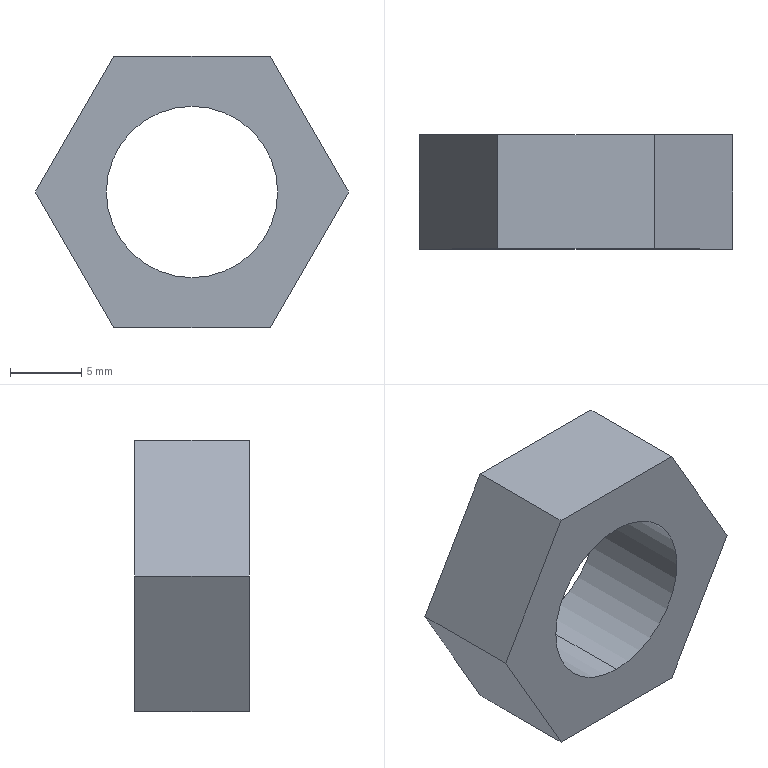Component | SolidWorks | M12Nut-1 | 1 solid | 10 faces | box 21.94 x 8 x 19 mm | volume 1596 mm3 | plane 8 | cylinder 2 | commonest cylinder face diameters 12 x2 | material #45
build123d program:
from build123d import *

# Parameters (mm, degrees)
BOSS_EXTRUDE1_DEPTH = 4
M12_TAPPED_HOLE1_D  = 12


with BuildPart() as part:
    # Sketch1 → Boss-Extrude1 (new, symmetric)
    with BuildSketch(Plane(origin=(0, 0, 0), x_dir=(1, 0, 0), z_dir=(0, 1, 0))):
        Polygon((5.485, 9.5), (-5.485, 9.5), (-10.97, 0), (-5.485, -9.5), (5.485, -9.5), (10.97, 0), align=None)
    extrude(amount=BOSS_EXTRUDE1_DEPTH, both=True)

    # M12 Tapped Hole1 (through all)
    with Locations(Plane(origin=(0, 4, 0), x_dir=(1, 0, 0), z_dir=(0, 1, 0))):
        with Locations((0, 0)):
            Hole(M12_TAPPED_HOLE1_D / 2)


solid = part.part

# Placed as in the assembly
solid = solid.moved(Location((40, -11.5, 60), (0, 0, 0)))
STEP:
#1=CARTESIAN_POINT('',(1.575,-0.6102,2.126));
#2=VERTEX_POINT('',#1);
#3=CARTESIAN_POINT('',(1.575,-0.6102,2.598));
#4=VERTEX_POINT('',#3);
#5=CARTESIAN_POINT('',(1.575,-0.6102,2.362));
#6=DIRECTION('',(0.,1.,0.));
#7=DIRECTION('',(0.,0.,1.));
#8=AXIS2_PLACEMENT_3D('',#5,#6,#7);
#9=CIRCLE('',#8,0.2362);
#10=EDGE_CURVE('',#2,#4,#9,.T.);
#11=ORIENTED_EDGE('',*,*,#10,.F.);
#12=CARTESIAN_POINT('',(1.575,-0.2953,2.126));
#13=VERTEX_POINT('',#12);
#14=CARTESIAN_POINT('',(1.575,-0.2953,2.126));
#15=DIRECTION('',(0.,1.,0.));
#16=VECTOR('',#15,39.37);
#17=LINE('',#14,#16);
#18=EDGE_CURVE('',#2,#13,#17,.T.);
#19=ORIENTED_EDGE('',*,*,#18,.T.);
#20=CARTESIAN_POINT('',(1.575,-0.2953,2.598));
#21=VERTEX_POINT('',#20);
#22=CARTESIAN_POINT('',(1.575,-0.2953,2.362));
#23=DIRECTION('',(0.,1.,0.));
#24=DIRECTION('',(0.,0.,1.));
#25=AXIS2_PLACEMENT_3D('',#22,#23,#24);
#26=CIRCLE('',#25,0.2362);
#27=EDGE_CURVE('',#13,#21,#26,.T.);
#28=ORIENTED_EDGE('',*,*,#27,.T.);
#29=CARTESIAN_POINT('',(1.575,-0.2953,2.598));
#30=DIRECTION('',(0.,1.,0.));
#31=VECTOR('',#30,39.37);
#32=LINE('',#29,#31);
#33=EDGE_CURVE('',#4,#21,#32,.T.);
#34=ORIENTED_EDGE('',*,*,#33,.F.);
#35=EDGE_LOOP('',(#11,#19,#28,#34));
#36=FACE_OUTER_BOUND('',#35,.T.);
#37=CARTESIAN_POINT('',(1.575,-0.2953,2.362));
#38=DIRECTION('',(0.,1.,0.));
#39=DIRECTION('',(0.,0.,1.));
#40=AXIS2_PLACEMENT_3D('',#37,#38,#39);
#41=CYLINDRICAL_SURFACE('',#40,0.2362);
#42=ADVANCED_FACE('',(#36),#41,.F.);
#43=CARTESIAN_POINT('',(2.007,-0.6102,2.362));
#44=VERTEX_POINT('',#43);
#45=CARTESIAN_POINT('',(1.791,-0.6102,1.988));
#46=VERTEX_POINT('',#45);
#47=CARTESIAN_POINT('',(2.007,-0.6102,2.362));
#48=DIRECTION('',(-0.5,0.,-0.866));
#49=VECTOR('',#48,39.37);
#50=LINE('',#47,#49);
#51=EDGE_CURVE('',#44,#46,#50,.T.);
#52=ORIENTED_EDGE('',*,*,#51,.T.);
#53=CARTESIAN_POINT('',(1.791,-0.2953,1.988));
#54=VERTEX_POINT('',#53);
#55=CARTESIAN_POINT('',(1.791,-0.2953,1.988));
#56=DIRECTION('',(0.,-1.,0.));
#57=VECTOR('',#56,39.37);
#58=LINE('',#55,#57);
#59=EDGE_CURVE('',#54,#46,#58,.T.);
#60=ORIENTED_EDGE('',*,*,#59,.F.);
#61=CARTESIAN_POINT('',(2.007,-0.2953,2.362));
#62=VERTEX_POINT('',#61);
#63=CARTESIAN_POINT('',(2.007,-0.2953,2.362));
#64=DIRECTION('',(-0.5,0.,-0.866));
#65=VECTOR('',#64,39.37);
#66=LINE('',#63,#65);
#67=EDGE_CURVE('',#62,#54,#66,.T.);
#68=ORIENTED_EDGE('',*,*,#67,.F.);
#69=CARTESIAN_POINT('',(2.007,-0.2953,2.362));
#70=DIRECTION('',(0.,-1.,0.));
#71=VECTOR('',#70,39.37);
#72=LINE('',#69,#71);
#73=EDGE_CURVE('',#62,#44,#72,.T.);
#74=ORIENTED_EDGE('',*,*,#73,.T.);
#75=EDGE_LOOP('',(#52,#60,#68,#74));
#76=FACE_OUTER_BOUND('',#75,.T.);
#77=CARTESIAN_POINT('',(2.007,-0.2953,2.362));
#78=DIRECTION('',(-0.866,0.,0.5));
#79=DIRECTION('',(0.5,0.,0.866));
#80=AXIS2_PLACEMENT_3D('',#77,#78,#79);
#81=PLANE('',#80);
#82=ADVANCED_FACE('',(#76),#81,.F.);
#83=CARTESIAN_POINT('',(1.359,-0.6102,1.988));
#84=VERTEX_POINT('',#83);
#85=CARTESIAN_POINT('',(1.791,-0.6102,1.988));
#86=DIRECTION('',(-1.,0.,0.));
#87=VECTOR('',#86,39.37);
#88=LINE('',#85,#87);
#89=EDGE_CURVE('',#46,#84,#88,.T.);
#90=ORIENTED_EDGE('',*,*,#89,.T.);
#91=CARTESIAN_POINT('',(1.359,-0.2953,1.988));
#92=VERTEX_POINT('',#91);
#93=CARTESIAN_POINT('',(1.359,-0.2953,1.988));
#94=DIRECTION('',(0.,-1.,0.));
#95=VECTOR('',#94,39.37);
#96=LINE('',#93,#95);
#97=EDGE_CURVE('',#92,#84,#96,.T.);
#98=ORIENTED_EDGE('',*,*,#97,.F.);
#99=CARTESIAN_POINT('',(1.791,-0.2953,1.988));
#100=DIRECTION('',(-1.,0.,0.));
#101=VECTOR('',#100,39.37);
#102=LINE('',#99,#101);
#103=EDGE_CURVE('',#54,#92,#102,.T.);
#104=ORIENTED_EDGE('',*,*,#103,.F.);
#105=ORIENTED_EDGE('',*,*,#59,.T.);
#106=EDGE_LOOP('',(#90,#98,#104,#105));
#107=FACE_OUTER_BOUND('',#106,.T.);
#108=CARTESIAN_POINT('',(1.791,-0.2953,1.988));
#109=DIRECTION('',(0.,0.,1.));
#110=DIRECTION('',(1.,0.,-0.));
#111=AXIS2_PLACEMENT_3D('',#108,#109,#110);
#112=PLANE('',#111);
#113=ADVANCED_FACE('',(#107),#112,.F.);
#114=CARTESIAN_POINT('',(1.143,-0.6102,2.362));
#115=VERTEX_POINT('',#114);
#116=CARTESIAN_POINT('',(1.359,-0.6102,1.988));
#117=DIRECTION('',(-0.5,0.,0.866));
#118=VECTOR('',#117,39.37);
#119=LINE('',#116,#118);
#120=EDGE_CURVE('',#84,#115,#119,.T.);
#121=ORIENTED_EDGE('',*,*,#120,.T.);
#122=CARTESIAN_POINT('',(1.143,-0.2953,2.362));
#123=VERTEX_POINT('',#122);
#124=CARTESIAN_POINT('',(1.143,-0.2953,2.362));
#125=DIRECTION('',(0.,-1.,0.));
#126=VECTOR('',#125,39.37);
#127=LINE('',#124,#126);
#128=EDGE_CURVE('',#123,#115,#127,.T.);
#129=ORIENTED_EDGE('',*,*,#128,.F.);
#130=CARTESIAN_POINT('',(1.359,-0.2953,1.988));
#131=DIRECTION('',(-0.5,0.,0.866));
#132=VECTOR('',#131,39.37);
#133=LINE('',#130,#132);
#134=EDGE_CURVE('',#92,#123,#133,.T.);
#135=ORIENTED_EDGE('',*,*,#134,.F.);
#136=ORIENTED_EDGE('',*,*,#97,.T.);
#137=EDGE_LOOP('',(#121,#129,#135,#136));
#138=FACE_OUTER_BOUND('',#137,.T.);
#139=CARTESIAN_POINT('',(1.359,-0.2953,1.988));
#140=DIRECTION('',(0.866,0.,0.5));
#141=DIRECTION('',(0.5,0.,-0.866));
#142=AXIS2_PLACEMENT_3D('',#139,#140,#141);
#143=PLANE('',#142);
#144=ADVANCED_FACE('',(#138),#143,.F.);
#145=CARTESIAN_POINT('',(1.359,-0.6102,2.736));
#146=VERTEX_POINT('',#145);
#147=CARTESIAN_POINT('',(1.143,-0.6102,2.362));
#148=DIRECTION('',(0.5,0.,0.866));
#149=VECTOR('',#148,39.37);
#150=LINE('',#147,#149);
#151=EDGE_CURVE('',#115,#146,#150,.T.);
#152=ORIENTED_EDGE('',*,*,#151,.T.);
#153=CARTESIAN_POINT('',(1.359,-0.2953,2.736));
#154=VERTEX_POINT('',#153);
#155=CARTESIAN_POINT('',(1.359,-0.2953,2.736));
#156=DIRECTION('',(0.,-1.,0.));
#157=VECTOR('',#156,39.37);
#158=LINE('',#155,#157);
#159=EDGE_CURVE('',#154,#146,#158,.T.);
#160=ORIENTED_EDGE('',*,*,#159,.F.);
#161=CARTESIAN_POINT('',(1.143,-0.2953,2.362));
#162=DIRECTION('',(0.5,0.,0.866));
#163=VECTOR('',#162,39.37);
#164=LINE('',#161,#163);
#165=EDGE_CURVE('',#123,#154,#164,.T.);
#166=ORIENTED_EDGE('',*,*,#165,.F.);
#167=ORIENTED_EDGE('',*,*,#128,.T.);
#168=EDGE_LOOP('',(#152,#160,#166,#167));
#169=FACE_OUTER_BOUND('',#168,.T.);
#170=CARTESIAN_POINT('',(1.143,-0.2953,2.362));
#171=DIRECTION('',(0.866,0.,-0.5));
#172=DIRECTION('',(-0.5,0.,-0.866));
#173=AXIS2_PLACEMENT_3D('',#170,#171,#172);
#174=PLANE('',#173);
#175=ADVANCED_FACE('',(#169),#174,.F.);
#176=CARTESIAN_POINT('',(1.791,-0.6102,2.736));
#177=VERTEX_POINT('',#176);
#178=CARTESIAN_POINT('',(1.359,-0.6102,2.736));
#179=DIRECTION('',(1.,0.,-0.));
#180=VECTOR('',#179,39.37);
#181=LINE('',#178,#180);
#182=EDGE_CURVE('',#146,#177,#181,.T.);
#183=ORIENTED_EDGE('',*,*,#182,.T.);
#184=CARTESIAN_POINT('',(1.791,-0.2953,2.736));
#185=VERTEX_POINT('',#184);
#186=CARTESIAN_POINT('',(1.791,-0.2953,2.736));
#187=DIRECTION('',(0.,-1.,0.));
#188=VECTOR('',#187,39.37);
#189=LINE('',#186,#188);
#190=EDGE_CURVE('',#185,#177,#189,.T.);
#191=ORIENTED_EDGE('',*,*,#190,.F.);
#192=CARTESIAN_POINT('',(1.359,-0.2953,2.736));
#193=DIRECTION('',(1.,0.,-0.));
#194=VECTOR('',#193,39.37);
#195=LINE('',#192,#194);
#196=EDGE_CURVE('',#154,#185,#195,.T.);
#197=ORIENTED_EDGE('',*,*,#196,.F.);
#198=ORIENTED_EDGE('',*,*,#159,.T.);
#199=EDGE_LOOP('',(#183,#191,#197,#198));
#200=FACE_OUTER_BOUND('',#199,.T.);
#201=CARTESIAN_POINT('',(1.359,-0.2953,2.736));
#202=DIRECTION('',(-0.,0.,-1.));
#203=DIRECTION('',(-1.,0.,0.));
#204=AXIS2_PLACEMENT_3D('',#201,#202,#203);
#205=PLANE('',#204);
#206=ADVANCED_FACE('',(#200),#205,.F.);
#207=CARTESIAN_POINT('',(1.791,-0.6102,2.736));
#208=DIRECTION('',(0.5,0.,-0.866));
#209=VECTOR('',#208,39.37);
#210=LINE('',#207,#209);
#211=EDGE_CURVE('',#177,#44,#210,.T.);
#212=ORIENTED_EDGE('',*,*,#211,.T.);
#213=ORIENTED_EDGE('',*,*,#73,.F.);
#214=CARTESIAN_POINT('',(1.791,-0.2953,2.736));
#215=DIRECTION('',(0.5,0.,-0.866));
#216=VECTOR('',#215,39.37);
#217=LINE('',#214,#216);
#218=EDGE_CURVE('',#185,#62,#217,.T.);
#219=ORIENTED_EDGE('',*,*,#218,.F.);
#220=ORIENTED_EDGE('',*,*,#190,.T.);
#221=EDGE_LOOP('',(#212,#213,#219,#220));
#222=FACE_OUTER_BOUND('',#221,.T.);
#223=CARTESIAN_POINT('',(1.791,-0.2953,2.736));
#224=DIRECTION('',(-0.866,0.,-0.5));
#225=DIRECTION('',(-0.5,0.,0.866));
#226=AXIS2_PLACEMENT_3D('',#223,#224,#225);
#227=PLANE('',#226);
#228=ADVANCED_FACE('',(#222),#227,.F.);
#229=CARTESIAN_POINT('',(1.575,-0.2953,2.362));
#230=DIRECTION('',(0.,1.,0.));
#231=DIRECTION('',(0.,0.,1.));
#232=AXIS2_PLACEMENT_3D('',#229,#230,#231);
#233=CIRCLE('',#232,0.2362);
#234=EDGE_CURVE('',#21,#13,#233,.T.);
#235=ORIENTED_EDGE('',*,*,#234,.F.);
#236=ORIENTED_EDGE('',*,*,#27,.F.);
#237=EDGE_LOOP('',(#235,#236));
#238=FACE_BOUND('',#237,.T.);
#239=ORIENTED_EDGE('',*,*,#67,.T.);
#240=ORIENTED_EDGE('',*,*,#103,.T.);
#241=ORIENTED_EDGE('',*,*,#134,.T.);
#242=ORIENTED_EDGE('',*,*,#165,.T.);
#243=ORIENTED_EDGE('',*,*,#196,.T.);
#244=ORIENTED_EDGE('',*,*,#218,.T.);
#245=EDGE_LOOP('',(#239,#240,#241,#242,#243,#244));
#246=FACE_OUTER_BOUND('',#245,.T.);
#247=CARTESIAN_POINT('',(1.575,-0.2953,2.362));
#248=DIRECTION('',(0.,1.,0.));
#249=DIRECTION('',(0.,0.,1.));
#250=AXIS2_PLACEMENT_3D('',#247,#248,#249);
#251=PLANE('',#250);
#252=ADVANCED_FACE('',(#238,#246),#251,.T.);
#253=CARTESIAN_POINT('',(1.575,-0.6102,2.362));
#254=DIRECTION('',(0.,1.,0.));
#255=DIRECTION('',(0.,0.,1.));
#256=AXIS2_PLACEMENT_3D('',#253,#254,#255);
#257=CIRCLE('',#256,0.2362);
#258=EDGE_CURVE('',#4,#2,#257,.T.);
#259=ORIENTED_EDGE('',*,*,#258,.T.);
#260=ORIENTED_EDGE('',*,*,#10,.T.);
#261=EDGE_LOOP('',(#259,#260));
#262=FACE_BOUND('',#261,.T.);
#263=ORIENTED_EDGE('',*,*,#51,.F.);
#264=ORIENTED_EDGE('',*,*,#211,.F.);
#265=ORIENTED_EDGE('',*,*,#182,.F.);
#266=ORIENTED_EDGE('',*,*,#151,.F.);
#267=ORIENTED_EDGE('',*,*,#120,.F.);
#268=ORIENTED_EDGE('',*,*,#89,.F.);
#269=EDGE_LOOP('',(#263,#264,#265,#266,#267,#268));
#270=FACE_OUTER_BOUND('',#269,.T.);
#271=CARTESIAN_POINT('',(1.575,-0.6102,2.362));
#272=DIRECTION('',(0.,1.,0.));
#273=DIRECTION('',(0.,0.,1.));
#274=AXIS2_PLACEMENT_3D('',#271,#272,#273);
#275=PLANE('',#274);
#276=ADVANCED_FACE('',(#262,#270),#275,.F.);
#277=ORIENTED_EDGE('',*,*,#18,.F.);
#278=ORIENTED_EDGE('',*,*,#258,.F.);
#279=ORIENTED_EDGE('',*,*,#33,.T.);
#280=ORIENTED_EDGE('',*,*,#234,.T.);
#281=EDGE_LOOP('',(#277,#278,#279,#280));
#282=FACE_OUTER_BOUND('',#281,.T.);
#283=CARTESIAN_POINT('',(1.575,-0.2953,2.362));
#284=DIRECTION('',(0.,1.,0.));
#285=DIRECTION('',(0.,0.,1.));
#286=AXIS2_PLACEMENT_3D('',#283,#284,#285);
#287=CYLINDRICAL_SURFACE('',#286,0.2362);
#288=ADVANCED_FACE('',(#282),#287,.F.);
#289=CLOSED_SHELL('',(#42,#82,#113,#144,#175,#206,#228,#252,#276,#288));
#290=MANIFOLD_SOLID_BREP('',#289);
#291=CARTESIAN_POINT('',(0.,0.,0.));
#292=DIRECTION('',(0.,0.,1.));
#293=DIRECTION('',(1.,0.,0.));
#294=AXIS2_PLACEMENT_3D('',#291,#292,#293);
#295=(LENGTH_UNIT()NAMED_UNIT(*)SI_UNIT($,.METRE.));
#296=LENGTH_MEASURE_WITH_UNIT(LENGTH_MEASURE(0.0254),#295);
#297=DIMENSIONAL_EXPONENTS(1.,0.,0.,0.,0.,0.,0.);
#298=(CONVERSION_BASED_UNIT('',#296)LENGTH_UNIT()NAMED_UNIT(#297));
#299=UNCERTAINTY_MEASURE_WITH_UNIT(LENGTH_MEASURE(0.00001),#298,'','');
#300=(NAMED_UNIT(*)PLANE_ANGLE_UNIT()SI_UNIT($,.RADIAN.));
#301=(NAMED_UNIT(*)SI_UNIT($,.STERADIAN.)SOLID_ANGLE_UNIT());
#302=(GEOMETRIC_REPRESENTATION_CONTEXT(3)GLOBAL_UNCERTAINTY_ASSIGNED_CONTEXT((#299))GLOBAL_UNIT_ASSIGNED_CONTEXT((#298,#300,#301))REPRESENTATION_CONTEXT('',''));
#303=ADVANCED_BREP_SHAPE_REPRESENTATION('',(#290,#294),#302);
#304=COLOUR_RGB('',0.7922,0.8196,0.9333);
#305=FILL_AREA_STYLE_COLOUR('',#304);
#306=FILL_AREA_STYLE('',(#305));
#307=SURFACE_STYLE_FILL_AREA(#306);
#308=SURFACE_SIDE_STYLE('',(#307));
#309=SURFACE_STYLE_USAGE(.BOTH.,#308);
#310=PRESENTATION_STYLE_ASSIGNMENT((#309));
#311=STYLED_ITEM('',(#310),#290);
#312=PRESENTATION_LAYER_ASSIGNMENT('','',(#311));
#313=(LENGTH_UNIT()NAMED_UNIT(*)SI_UNIT($,.METRE.));
#314=LENGTH_MEASURE_WITH_UNIT(LENGTH_MEASURE(0.0254),#313);
#315=DIMENSIONAL_EXPONENTS(1.,0.,0.,0.,0.,0.,0.);
#316=(CONVERSION_BASED_UNIT('',#314)LENGTH_UNIT()NAMED_UNIT(#315));
#317=UNCERTAINTY_MEASURE_WITH_UNIT(LENGTH_MEASURE(0.00001),#316,'','');
#318=(NAMED_UNIT(*)PLANE_ANGLE_UNIT()SI_UNIT($,.RADIAN.));
#319=(NAMED_UNIT(*)SI_UNIT($,.STERADIAN.)SOLID_ANGLE_UNIT());
#320=(GEOMETRIC_REPRESENTATION_CONTEXT(3)GLOBAL_UNCERTAINTY_ASSIGNED_CONTEXT((#317))GLOBAL_UNIT_ASSIGNED_CONTEXT((#316,#318,#319))REPRESENTATION_CONTEXT('',''));
#321=MECHANICAL_DESIGN_GEOMETRIC_PRESENTATION_REPRESENTATION('',(#311),#320);